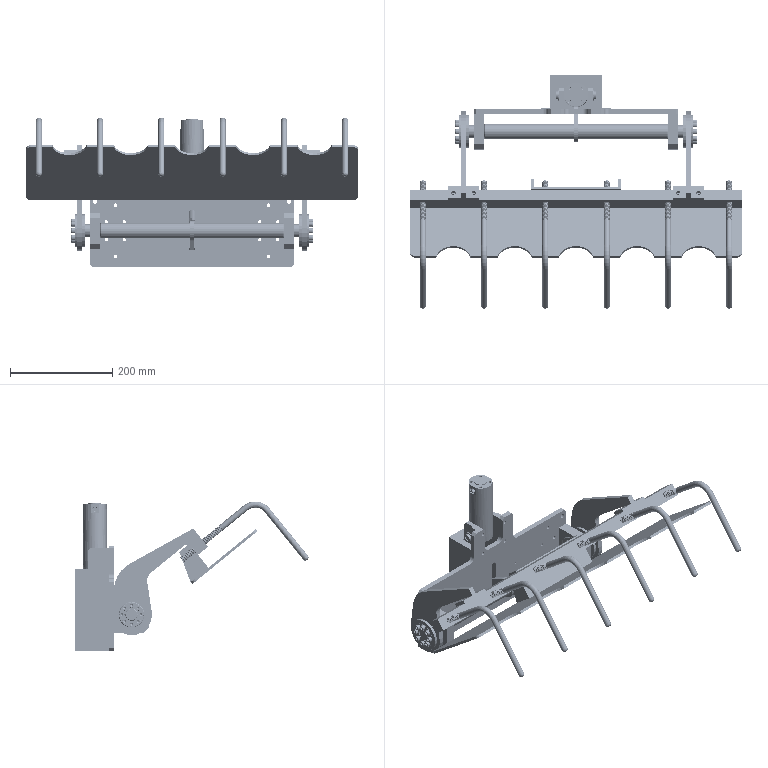Assembly | SolidWorks | mm | 42 component files | 42 solids | 5395 faces | box 650 x 456.8 x 291.75 mm | volume 2823567 mm3 | cone 3668 | cylinder 982 | plane 525 | torus 172 | sphere 48 | commonest cylinder face diameters 12 x614 10 x42 6 x32 6.012 x32 6.8 x24 9 x20 14 x20 6.5 x16
Bill of materials:
000504Y000006205 | 2 |  | Annular ring assembly: an outer ring and an inner ring on the same axis, with a single row of spherical balls between them; no cage or shields visible. The shape matches an open radial ball bearing.
CG1UN40-50CylinderBlock | 1 |  | Upright cylindrical body. The top face has a raised circular boss and four small holes around it. A short boss with a round port sits on the side near the top. Near the bottom, two coaxial tubular stubs stick out on opposite sides, each with a thin flange ring. There is a circumferential seam line near the base.
CG1UN40-50Nut | 1 |  | Hexagonal nut-like body with a large plain round through bore and chamfered corners on both faces.
CG1UN40-50Piston | 1 |  | Headed pin: a thin flat circular head on a long cylindrical shank. The shank steps down to a smaller diameter near the free end, and a small notch or flat sits at the step.
OT-0100-001(HookSeat) | 1 | Plain Carbon Steel | Long straight bar with a square cross-section. Six evenly spaced holes run along one face, and four smaller holes sit in pairs near each end on an adjacent face.
OT-0100-002(Hook) | 6 | AISI 304 | Round rod bent into a wide L or V shape with a rounded bend. One leg ends in a section with thread-like ridges; the other leg is plain with a rounded end.
OT-0100-003(SwingRod) | 2 | Plain Carbon Steel | Flat lever or arm made from plate. A rounded end has a circular hole with a raised hub ring around it. The arm angles away and ends in a small rectangular block or tab that is perpendicular to the plate and has two holes.
OT-0100-004(BasePlate) | 1 |  | Flat rectangular plate with two raised tabs on one long edge, forming a U-shaped notch between them. It has a central elongated slot, many round holes in roughly symmetric groups toward each end, and chamfered corners.
OT-0100-005(RotatingShaft) | 1 | Plain Carbon Steel | Long stepped round shaft with smaller-diameter steps at both ends. Near mid-length, a flat lever arm with a hub sticks out sideways and ends in a rounded tip with a small hole.
OT-0100-006(MaterialStopBlock) | 1 | AISI 304 | Thin rectangular plate with five evenly spaced semicircular notches along one long edge and rounded corners. A narrower rectangular tab with two holes stands at an angle to the plate near the middle of the opposite edge.
OT-0100-007(BearingHousing) | 2 | Plain Carbon Steel | Square block with a large round through bore and one chamfered corner. A thin groove or recess ring runs inside the bore.
OT-0100-008(LiveHinge) | 1 | Plain Carbon Steel | Rectangular block shaped like a clevis. An axial round bore enters the top face, a through slot from the bottom splits the lower portion into two legs, and a cross hole passes through both legs. The bottom edges are chamfered.
OT-0100-009(TrunnionSeat) | 2 | Plain Carbon Steel | Rectangular plate-like block with a step along one edge, one large round through-hole in the main face, two angled-chamfered corners on the edge opposite the step, and two small holes in one narrow side face.
OT-0100-029(CylinderGuard) | 1 |  | Thin-walled rectangular box-like housing, open on one face, with a U-shaped slot (rounded end) cut into the top wall and two small flat tabs with round holes sticking out from opposite sides.
OT-0200-012(PinShaft) | 1 | Plain Carbon Steel | Headed cylindrical pin: a larger-diameter short disc-shaped head on a long plain cylindrical shank, with a narrow circumferential groove near the flat far end.
000102Z000060016 | 16 |  | Cap-screw-like fastener: a cylindrical head with a rounded top edge on an externally threaded shank, with a short unthreaded neck/fillet under the head and a chamfered tip.
Z24X50X20LockingAssembly | 2 |  | Thick plain annular ring (spacer/washer-like) with a central through-bore and small chamfers on its outer edges.
Mates:
1. concentric | OT-0100-007(BearingHousing)-1 face at (5, 35, 0) dir (1, 0, 0) r 26 | OT-0100-005(RotatingShaft)-1 face at (410, 35, 0) dir (1, 0, 0) r 12.5
2. coincident | OT-0100-007(BearingHousing)-1 face at (20, 0, 0) dir (1, 0, 0) | OT-0100-005(RotatingShaft)-1 face at (20, 30.501, -11.662) dir (-1, 0, 0)
3. concentric | OT-0100-005(RotatingShaft)-1 face at (410, 35, 0) dir (1, 0, 0) r 15 | OT-0100-007(BearingHousing)-2 face at (395, 35, 0) dir (-1, 0, 0) r 26
4. coincident | OT-0100-005(RotatingShaft)-1 face at (380, 29.961, -13.062) dir (1, 0, 0) | OT-0100-007(BearingHousing)-2 face at (380, 0, 0) dir (-1, 0, 0)
5. coincident | OT-0100-007(BearingHousing)-1 face at (20, 70, 35) dir (0, 1, 0) | OT-0100-007(BearingHousing)-2 face at (380, 70, -35) dir (0, 1, 0)
6. concentric | OT-0100-005(RotatingShaft)-1 face at (-30, 35, 0) dir (1, 0, 0) r 12 | OT-0100-003(SwingRod)-1 face at (-30, 35, 0) dir (1, 0, 0) r 25
7. coincident | OT-0100-005(RotatingShaft)-1 face at (-30, 35, 0) dir (-1, 0, 0) | OT-0100-003(SwingRod)-1 face at (-30, 35, 0) dir (-1, 0, 0)
8. coincident | OT-0100-003(SwingRod)-1 face at (-50.001, -98.775, 152.513) dir (0, -0.6306, -0.7761) | OT-0100-001(HookSeat)-1 face at (-125, -79.373, 136.747) dir (0, 0.6306, 0.7761)
9. coincident | OT-0100-003(SwingRod)-1 face at (-50.001, -80.634, 135.195) dir (0, -0.7761, 0.6306) | OT-0100-001(HookSeat)-1 face at (200, -87.256, 127.046) dir (0, 0.7761, -0.6306)
10. concentric | OT-0100-003(SwingRod)-1 face at (-40, -135.741, 87.2) dir (0, 0.6306, 0.7761) r 4.5 | OT-0100-001(HookSeat)-1 face at (-40, -89.074, 144.63) dir (0, 0.6306, 0.7761) r 3.4
11. concentric | OT-0100-005(RotatingShaft)-1 face at (410, 35, 0) dir (1, 0, 0) r 15 | OT-0100-003(SwingRod)-2 face at (410, 35, 0) dir (1, 0, 0) r 25
12. concentric | OT-0100-001(HookSeat)-1 face at (400, -89.074, 144.63) dir (0, 0.6306, 0.7761) r 3.4 | OT-0100-003(SwingRod)-2 face at (400, -135.741, 87.2) dir (0, 0.6306, 0.7761) r 4.5
13. concentric | OT-0100-001(HookSeat)-1 face at (440, -89.074, 144.63) dir (0, 0.6306, 0.7761) r 3.4 | OT-0100-003(SwingRod)-2 face at (440, -135.741, 87.2) dir (0, 0.6306, 0.7761) r 4.5
14. concentric | OT-0100-001(HookSeat)-1 face at (-100, -106.658, 142.813) dir (0, 0.7761, -0.6306) r 6.25 | OT-0100-002(Hook)-1 face at (-100, -188.146, 209.029) dir (0, 0.7761, -0.6306) r 6
15. parallel | OT-0100-001(HookSeat)-1 face at (-125, -79.373, 136.747) dir (-1, 0, 0) | OT-0100-002(Hook)-1 plane at (-100, -211.429, 227.948) dir (1, 0, 0)
16. distance | OT-0100-002(Hook)-1 face at (-100, -63.973, 108.127) dir (0, 0.7761, -0.6306) | OT-0100-001(HookSeat)-1 face at (200, -87.256, 127.046) dir (0, 0.7761, -0.6306)
17. concentric | OT-0100-001(HookSeat)-1 face at (140, -106.658, 142.813) dir (0, 0.7761, -0.6306) r 6.25 | OT-0100-006(MaterialStopBlock)-1 face at (140, -180.386, 202.723) dir (0, 0.7761, -0.6306) r 6.5
18. concentric | OT-0100-001(HookSeat)-1 face at (260, -106.658, 142.813) dir (0, 0.7761, -0.6306) r 6.25 | OT-0100-006(MaterialStopBlock)-1 face at (260, -180.386, 202.723) dir (0, 0.7761, -0.6306) r 6.5
19. concentric | OT-0100-007(BearingHousing)-2 face at (395, 35, 0) dir (-1, 0, 0) r 26 | 000504Y000006205-1 face at (298.393, 35, 0) dir (-1, 0, 0) r 26
20. coincident | OT-0100-007(BearingHousing)-2 face at (380, 0, 0) dir (-1, 0, 0) | 000504Y000006205-1 face at (380, 56.5, 0) dir (-1, 0, 0)
21. concentric | OT-0100-007(BearingHousing)-1 face at (5, 35, 0) dir (1, 0, 0) r 26 | 000504Y000006205-2 face at (-76.607, 35, 0) dir (-1, 0, 0) r 12.5
22. coincident | OT-0100-007(BearingHousing)-1 face at (20, 0, 0) dir (1, 0, 0) | 000504Y000006205-2 face at (20, 61, 0) dir (1, 0, 0)
23. coincident | OT-0100-007(BearingHousing)-1 face at (20, 70, 35) dir (0, 1, 0) | OT-0100-004(BasePlate)-1 face at (136, 70, 80) dir (0, -1, 0)
24. concentric | OT-0100-007(BearingHousing)-1 face at (10, 70, -27.5) dir (0, 1, 0) r 3.4 | OT-0100-004(BasePlate)-1 face at (10, 80, -27.5) dir (0, -1, 0) r 4.5
25. concentric | OT-0100-007(BearingHousing)-1 face at (10, 70, 27.5) dir (0, 1, 0) r 3.4 | OT-0100-004(BasePlate)-1 face at (10, 80, 27.5) dir (0, -1, 0) r 4.5
26. concentric | CG1UN40-50CylinderBlock-1 face at (200, 106.5, 162.548) dir (0, 0.008055, 1) r 23.5 | CG1UN40-50Piston-1 face at (200, 105.69, 62.001) dir (0, 0.008055, 1) r 8
27. concentric | CG1UN40-50Piston-1 face at (200, 105.69, 62.001) dir (0, 0.008055, 1) r 8 | CG1UN40-50Nut-1 face at (200, 105.247, 7.003) dir (0, 0.008055, 1) r 7
28. distance | CG1UN40-50Nut-1 face at (200, 105.215, 3.003) dir (0, -0.008055, -1) | CG1UN40-50Piston-1 face at (198.296, 102.629, -11.476) dir (0, -0.008055, -1)
29. coincident | OT-0100-005(RotatingShaft)-1 face at (204, 35, 0) dir (1, 0, 0) | OT-0100-008(LiveHinge)-1 face at (204, 94.892, -36.915) dir (-1, 0, 0)
30. concentric | OT-0100-005(RotatingShaft)-1 face at (196, 104.973, -26.996) dir (1, 0, 0) r 5 | OT-0100-008(LiveHinge)-1 face at (210, 104.973, -26.996) dir (-1, 0, 0) r 5
31. concentric | CG1UN40-50Piston-1 face at (200, 105.211, 2.503) dir (0, 0.008055, 1) r 7 | OT-0100-008(LiveHinge)-1 face at (200, 105.215, 3.003) dir (0, 0.008055, 1) r 7
32. coincident | CG1UN40-50Nut-1 face at (200, 105.215, 3.003) dir (0, -0.008055, -1) | OT-0100-008(LiveHinge)-1 face at (190, 115.214, 2.923) dir (0, 0.008055, 1)
33. distance | CG1UN40-50Piston-1 face at (198.296, 102.629, -11.476) dir (0, -0.008055, -1) | CG1UN40-50CylinderBlock-1 face at (200, 123.903, 88.355) dir (0, -0.008055, -1)
34. coincident | OT-0100-004(BasePlate)-1 face at (136, 80, 80) dir (0, 1, 0) | OT-0100-009(TrunnionSeat)-1 face at (176, 80, 130.5) dir (0, -1, 0)
35. concentric | OT-0100-004(BasePlate)-1 face at (170, 69.999, 123) dir (0, 1, 0) r 3.5 | OT-0100-009(TrunnionSeat)-1 face at (170, 80, 123) dir (0, -1, 0) r 2.5
36. concentric | OT-0100-004(BasePlate)-1 face at (170, 69.999, 78) dir (0, 1, 0) r 3.5 | OT-0100-009(TrunnionSeat)-1 face at (170, 80, 78) dir (0, -1, 0) r 2.5
37. concentric | CG1UN40-50CylinderBlock-1 face at (172.625, 106, 100.5) dir (1, 0, 0) r 7 | OT-0100-009(TrunnionSeat)-1 face at (176, 106, 100.5) dir (-1, 0, 0) r 7
38. coincident | OT-0100-004(BasePlate)-1 face at (136, 80, 80) dir (0, 1, 0) | OT-0100-009(TrunnionSeat)-2 face at (224, 80, 70.5) dir (0, -1, 0)
39. concentric | OT-0100-004(BasePlate)-1 face at (230, 69.999, 78) dir (0, 1, 0) r 3.5 | OT-0100-009(TrunnionSeat)-2 face at (230, 80, 78) dir (0, -1, 0) r 2.5
40. concentric | OT-0100-004(BasePlate)-1 face at (230, 69.999, 123) dir (0, 1, 0) r 3.5 | OT-0100-009(TrunnionSeat)-2 face at (230, 80, 123) dir (0, -1, 0) r 2.5
41. concentric | OT-0100-003(SwingRod)-1 face at (-30, 35, 0) dir (1, 0, 0) r 25 | Z24X50X20LockingAssembly-1/Z24X50X20LockingAssembly-1 face at (-30, 35, 0) dir (1, 0, 0) r 25
42. coincident | OT-0100-003(SwingRod)-1 face at (-30, 35, 0) dir (-1, 0, 0) | Z24X50X20LockingAssembly-1/Z24X50X20LockingAssembly-1 face at (-30, 35, 0) dir (-1, 0, 0)
43. concentric | OT-0100-003(SwingRod)-2 face at (410, 35, 0) dir (1, 0, 0) r 25 | Z24X50X20LockingAssembly-2/Z24X50X20LockingAssembly-1 face at (430, 35, 0) dir (-1, 0, 0) r 25
44. coincident | OT-0100-003(SwingRod)-2 face at (430, 35, 0) dir (1, 0, 0) | Z24X50X20LockingAssembly-2/Z24X50X20LockingAssembly-1 face at (430, 35, 0) dir (1, 0, 0)
45. coincident | OT-0100-008(LiveHinge)-1 face at (190, 114.892, -37.076) dir (-1, 0, 0) | OT-0200-012(PinShaft)-1 face at (190, 104.973, -33.996) dir (1, 0, 0)
46. concentric | OT-0100-008(LiveHinge)-1 face at (210, 104.973, -26.996) dir (-1, 0, 0) r 5 | OT-0200-012(PinShaft)-1 face at (213, 104.973, -26.996) dir (1, 0, 0) r 5
47. angle | OT-0100-005(RotatingShaft)-1 plane at (200, 35, 0) dir (0, 0.3599, 0.933) | OT-0100-003(SwingRod)-1 face at (-15, -94.991, 157.17) dir (0, -0.6306, -0.7761)
48. coincident | OT-0100-001(HookSeat)-1 face at (200, -87.256, 127.046) dir (0, 0.7761, -0.6306) | OT-0100-006(MaterialStopBlock)-1 face at (112.5, -77.796, 138.688) dir (0, -0.7761, 0.6306)
49. coincident | OT-0100-004(BasePlate)-1 face at (136, 80, 80) dir (0, 1, 0) | OT-0100-029(CylinderGuard)-1 face at (200, 80, 10) dir (0, -1, 0)
50. coincident | OT-0100-004(BasePlate)-1 face at (400, 80, -70) dir (0, 0, -1) | OT-0100-029(CylinderGuard)-1 face at (150, 80, -70) dir (0, 0, -1)
51. coincident | OT-0100-004(BasePlate)-1 plane at (200, 70, -70) dir (-1, 0, 0) | OT-0100-029(CylinderGuard)-1 plane at (200, 145, 10) dir (1, 0, 0)
52. coincident | Z24X50X20LockingAssembly-1 face at (0, 20, 0) dir (0, 1, 0) | 000102Z000060016-1 face at (23.7, 20, 0) dir (0, -1, 0)
53. concentric | Z24X50X20LockingAssembly-1 face at (18.7, 20, 0) dir (0, 1, 0) r 3 | 000102Z000060016-1 face at (18.7, 127.416, 0) dir (0, 1, 0) r 5